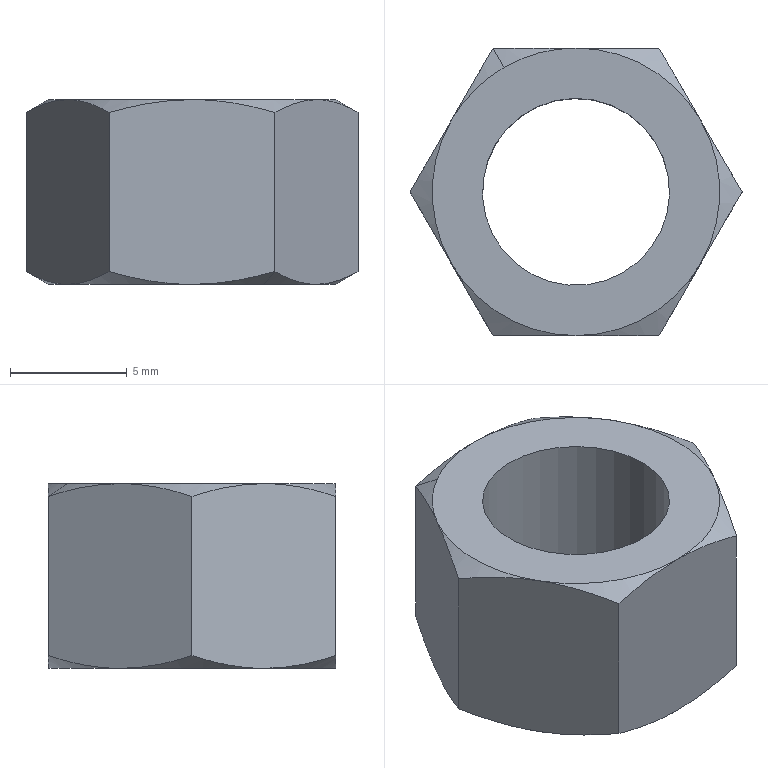Component | NX | HEX_NUT_M8_2 | 1 solid | 23 faces | volume 633 mm3 | cone 14 | plane 8 | cylinder 1 | commonest cylinder face diameters 8 x1